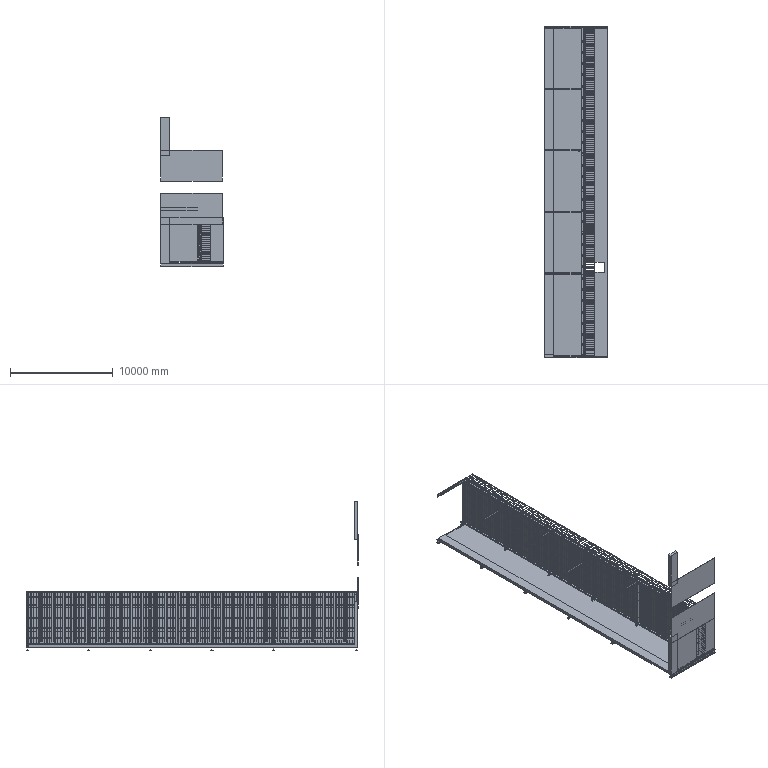Assembly | SolidWorks | mm | 472 component files | 530 solids | 11239 faces | box 6100 x 32341.42 x 14577.61 mm | volume 24746650782 mm3 | plane 7610 | cylinder 3629 | commonest cylinder face diameters 12 x1644 6 x1644 26 x76 2.667 x70 10 x58 20 x58 56 x44 14 x35
Bill of materials:
30X30X3-1100 | 16 |  | Long straight square hollow tube with rounded outer and inner corners and a uniform wall.
30X30X3-940 | 162 |  | Long straight square hollow tube with rounded corners and a uniform wall.
63#AngleIron | 20 |  | Long angle (L-section) profile with legs of roughly equal length, a root fillet and slightly rounded leg tips. A narrow gap splits the length into two collinear pieces.
8mTread | 4 |  | Thin flat rectangular plate or strip with no visible holes or edge features.
ChannelSteel | 29 |  | Long straight channel (C-section) with sloped inner flange faces, root fillets between web and flanges, and rounded flange tips.
ColorSteelTile | 1 |  | Thin sheet-metal-like strip with one end bent up 90 degrees into a flange, giving an L-shaped side profile. The flat part has one rectangular cutout and a row of small slots or holes along its length.
Corbel | 5 |  | Short piece of wide-flange H/I-section with parallel flanges, a central web and large root fillets.
H200X100-3600 | 6 |  | Long I-section beam that is deep relative to its flange width, with a thin web, thin parallel flanges and root fillets.
H250X125-3800 | 5 |  | Long, slender H-section member with wide parallel flanges, a thin web and root fillets.
H250X125-7375 | 8 |  | Long H-section profile with wide flanges, a thin web and root fillets. It is shown lying with the web horizontal, so it looks like a trough in the isometric view.
Mirror30X30X3-940 | 159 |  | Long straight square hollow tube with rounded corners and a uniform wall.
Mirror30X30X3-1100 | 14 |  | Long straight square hollow tube with rounded corners and a uniform wall.
Mirror30X30X3-7440 | 8 |  | Long, slender straight tube with a square hollow cross-section and rounded corners. The length shows small breaks or seams, so it looks like three collinear lengths.
Mirror30X30X3-3720-30 | 2 |  | Straight square hollow tube with rounded corners, shown as a long thin member with breaks or seams dividing it into three collinear segments.
OriginalColumn | 6 |  | Straight I-section beam (wide-flange-like profile) with a constant cross-section along its length.
30X30X3-3720-30 | 2 |  | Straight square hollow tube with rounded corners, shown as a long thin member with breaks or seams dividing it into three collinear segments.
30X30X3-7440 | 8 |  | Long, slender straight tube with a square hollow cross-section and rounded corners. The length shows small breaks or seams, so it looks like three collinear lengths.
Tread | 16 |  | Thin flat rectangular plate or sheet with no visible holes or cutouts.
Wall | 1 |  | L-shaped arrangement of thin flat bars: a long horizontal strip joined at one end to a short upright strip. Two rectangular plates, separated by a gap, project sideways from the upright.
Mates:
1. width | H250X125-3800-1 face at (2060.926, 805.154, 99) dir (0, -1, 0) | H250X125-3800-1 face at (2069.926, 930.154, 99) dir (0, 1, 0) | OriginalColumn-1 face at (4369.926, 977.654, -147.679) dir (0, 1, 0) | OriginalColumn-1 face at (4369.926, 757.654, -167.679) dir (0, -1, 0)
2. coincident | H200X100-3600-1 face at (1819.926, 851.904, 5050) dir (1, 0, 0) | H250X125-3800-1 face at (1819.926, 930.154, 99) dir (-1, 0, 0)
3. width | H200X100-3600-1 face at (1819.926, 805.154, 5029) dir (0, -1, 0) | H200X100-3600-1 face at (1819.926, 930.154, 5037) dir (0, 1, 0) | H250X125-3800-1 face at (1828.926, 930.154, 99) dir (0, 1, 0) | H250X125-3800-1 face at (1819.926, 805.154, 99) dir (0, -1, 0)
4. coincident | H200X100-3600-1 face at (1819.926, 805.154, 5279) dir (0, 0, 1) | H250X125-3800-1 face at (1841.926, 851.654, 5279) dir (0, 0, 1)
5. coincident | H250X125-3800-1 face at (2069.926, 805.154, 99) dir (1, 0, 0) | H250X125-7375-1 face at (2069.926, 805.154, 5154) dir (1, 0, 0)
6. coincident | H250X125-3800-1 face at (1819.926, 805.154, 99) dir (0, -1, 0) | H250X125-7375-1 face at (1841.926, 805.154, 5200.5) dir (0, 1, 0)
7. distance | ChannelSteel-1 face at (1912.304, -394.846, 164.5) dir (0, 1, 0) | H250X125-3800-1 face at (2060.926, 805.154, 99) dir (0, -1, 0)
8. coincident | H250X125-3800-1 face at (2069.926, 805.154, 99) dir (1, 0, 0) | 63#AngleIron-1 face at (2069.926, 805.154, 4696) dir (1, 0, 0)
9. coincident | H250X125-3800-1 face at (2060.926, 805.154, 99) dir (0, -1, 0) | 63#AngleIron-1 face at (2008.259, 805.154, 4756.333) dir (0, 1, 0)
10. coincident | H250X125-3800-1 face at (2069.926, 805.154, 99) dir (1, 0, 0) | assembly face at (2069.774, 874.154, 4042) dir (-1, 0, 0)
11. distance | assembly face at (3169.774, 880.154, 4042) dir (0, 1, 0) | H250X125-3800-1 face at (2069.926, 930.154, 99) dir (0, 1, 0)
12. distance | assembly face at (3169.774, 874.154, 4048) dir (0, 0, 1) | H250X125-3800-1 face at (1841.926, 851.654, 5279) dir (0, 0, 1)
13. coincident | ChannelSteel-1 face at (1912.304, -594.846, 164.5) dir (1, 0, 0) | Floor-1 face at (2069.774, 930.154, 2588) dir (-1, 0, 0)
14. coincident | H250X125-7375-1 face at (2069.926, 805.154, 5279) dir (0, 0, 1) | Floor-1 face at (2069.774, 930.154, 4098) dir (0, 0, 1)
15. coincident | H250X125-3800-1 face at (2069.926, 930.154, 99) dir (0, 1, 0) | Floor-1 face at (2069.774, 930.154, 2588) dir (0, 1, 0)
16. coincident | assembly face at (3169.774, 880.154, 4042) dir (0, 1, 0) | assembly face at (3169.774, 880.154, 322) dir (0, -1, 0)
17. coincident | assembly face at (3169.774, 874.154, 4048) dir (0, 0, 1) | assembly face at (3169.774, 886.154, 4048) dir (0, 0, 1)
18. coincident | OriginalColumn-1 face at (4369.926, 757.654, -167.679) dir (0, -1, 0) | assembly face at (3169.774, 717.654, -128) dir (0, 1, 0)
19. distance | OriginalColumn-2 face at (4369.926, -5098.346, -167.679) dir (0, 0, -1) | assembly face at (3169.774, -6458.346, -122) dir (0, 0, 1)
20. coincident | Tread-1 face at (2069.926, 8778.376, -4819.381) dir (-1, 0, 0) | H250X125-7375-15 face at (2019.774, 805.154, 99) dir (1, 0, 0)
21. coincident | OriginalColumn-1 face at (4369.926, 757.654, -147.679) dir (0, 0, 1) | Corbel-1 face at (1771.926, 833.654, -147.679) dir (0, 0, -1)
22. width | OriginalColumn-1 face at (4369.926, 977.654, -147.679) dir (0, 1, 0) | OriginalColumn-1 face at (4369.926, 757.654, -167.679) dir (0, -1, 0) | Corbel-1 face at (1819.926, 805.154, 352.321) dir (0, -1, 0) | Corbel-1 face at (1799.926, 930.154, 352.321) dir (0, 1, 0)
23. coincident | OriginalColumn-1 face at (-1730.074, 833.654, -449.679) dir (-1, 0, 0) | Wall-1 face at (-1730.074, 4663.226, -160.714) dir (-1, 0, 0)
24. coincident | OriginalColumn-1 face at (4369.926, 757.654, -147.679) dir (0, 0, 1) | Wall-1 face at (-830.074, 757.654, -147.679) dir (0, 0, -1)
25. distance | H250X125-7375-15 face at (2010.774, 805.154, 99) dir (0, 0, -1) | Tread-1 face at (2069.926, 890.154, 139) dir (0, 0, -1)
26. distance | H250X125-7375-16 face at (1841.926, 805.154, 158.5) dir (0, 0, -1) | OriginalColumn-1 face at (4369.926, 757.654, -147.679) dir (0, 0, 1)
27. distance | H250X125-3800-1 face at (1841.926, 851.654, 99) dir (0, 0, -1) | Tread-1 face at (2069.926, 890.154, 139) dir (0, 0, -1)
28. coincident | Railing-2-2/30X30X3-1100-3 face at (3169.926, -31194.846, 3843) dir (0, -1, 0) | 30X30X3-1100-3 face at (3169.926, -31194.846, 5273) dir (0, -1, 0)
29. coincident | Railing-2-2/30X30X3-3720-30-1 face at (3163.926, -31170.846, 5249) dir (0, 0, 1) | 30X30X3-1100-3 face at (3169.926, -31170.846, 5249) dir (0, 0, -1)
30. coincident | Railing-2-2/30X30X3-3720-30-1 face at (3169.926, -31170.846, 5249) dir (1, 0, 0) | 30X30X3-1100-3 face at (3169.926, -31170.846, 5255) dir (1, 0, 0)
31. coincident | Railing-2-2/30X30X3-940-16 face at (3139.926, -31194.846, 3648) dir (0, -1, 0) | 30X30X3-940-1 face at (3139.926, -31194.846, 3908) dir (0, -1, 0)
32. coincident | Railing-2-2/30X30X3-3720-30-2 face at (2199.926, -31170.846, 5249) dir (1, 0, 0) | 30X30X3-940-1 face at (2199.926, -31170.846, 3890) dir (-1, 0, 0)
33. coincident | H200X100-3600-6 face at (-1730.074, -29148.096, 5050) dir (-1, 0, 0) | Wall-1 face at (-1730.074, 4663.226, -160.714) dir (-1, 0, 0)
34. coincident | Tread-1 face at (2069.926, 8778.376, -4819.381) dir (-1, 0, 0) | H250X125-7375-16 face at (2069.926, 805.154, 99) dir (1, 0, 0)
35. lock | H250X125-3800-6 reference at (0, 0, 0) dir (1, 0, 0) | 30X30X3-1100-3 reference at (0, 0, 0) dir (1, 0, 0)
36. coincident | H250X125-3800-1 face at (2069.926, 805.154, 99) dir (1, 0, 0) | Railing-6/30X30X3-1100-1 face at (2069.926, 922.294, 5273) dir (-1, 0, 0)
37. coincident | H250X125-7375-4 face at (2069.926, -23194.846, 5154) dir (1, 0, 0) | 30X30X3-1100-3 face at (2069.926, -31170.846, 5255) dir (-1, 0, 0)
38. coincident | H250X125-7375-4 face at (2069.926, -23194.846, 5279) dir (0, 0, 1) | 30X30X3-1100-3 face at (3169.926, -31188.846, 5279) dir (0, 0, 1)
39. coincident | H250X125-7375-4 face at (1841.926, -31194.846, 5200.5) dir (0, -1, 0) | 30X30X3-1100-3 face at (3169.926, -31194.846, 5273) dir (0, -1, 0)
40. coincident | Railing-6/30X30X3-1100-3 face at (3169.926, -6547.706, 5279) dir (0, 0, 1) | 30X30X3-940-6 face at (3139.926, -6811.197, 5279) dir (0, 0, 1)
41. lock | H250X125-7375-4 reference at (0, 0, 0) dir (1, 0, 0) | 30X30X3-1100-3 reference at (0, 0, 0) dir (1, 0, 0)
42. coincident | H250X125-7375-19 face at (2069.926, -23194.846, 99) dir (1, 0, 0) | 8mTread-1 face at (2069.926, -13426.79, -4794.447) dir (-1, 0, 0)
43. coincident | Tread-76 edge at (2077.926, -17139.846, 139) dir (0, -1, 0) | 8mTread-1 edge at (2077.926, -23149.846, 139) dir (0, -1, 0)
44. distance | Tread-76 face at (2069.926, -23139.846, 139) dir (0, -1, 0) | 8mTread-1 face at (2069.926, -23149.846, 139) dir (0, 1, 0)
45. distance | H250X125-3800-1 face at (1841.926, 851.654, 99) dir (0, 0, -1) | ChannelSteel-1 vertex at (1894.378, -405.685, 164.5) dir (1, 0, 0)
46. lock | H250X125-3800-1 reference at (0, 0, 0) dir (1, 0, 0) | Railing-6/30X30X3-1100-1 reference at (0, 0, 0) dir (1, 0, 0)
47. lock | Railing-6/30X30X3-7440-1 reference at (0, 0, 0) dir (1, 0, 0) | 30X30X3-940-6 reference at (0, 0, 0) dir (1, 0, 0)
48. coincident | Mirror30X30X3-1100-1 face at (-381.487, 603.212, -30) dir (0, 0, -1) | Mirror30X30X3-7440-1 face at (7642.513, 597.212, -30) dir (0, 0, -1)
49. coincident | Mirror30X30X3-1100-1 face at (-357.487, 603.212, -6) dir (1, 0, 0) | Mirror30X30X3-7440-1 face at (-357.487, 597.212, -24) dir (-1, 0, 0)
50. coincident | Mirror30X30X3-1100-1 face at (-381.487, 603.212, -24) dir (0, 1, 0) | Mirror30X30X3-7440-1 face at (7642.513, 603.212, -24) dir (0, 1, 0)
51. coincident | Mirror30X30X3-1100-1 face at (-381.487, 603.212, -30) dir (0, 0, -1) | Mirror30X30X3-940-1 face at (-171.487, 573.212, -30) dir (0, 0, -1)
52. coincident | Mirror30X30X3-7440-1 face at (7642.513, 573.212, -6) dir (0, -1, 0) | Mirror30X30X3-940-1 face at (-171.487, 573.212, -24) dir (0, 1, 0)
53. coincident | Mirror30X30X3-1100-1 face at (-381.487, 603.212, -30) dir (0, 0, -1) | Mirror30X30X3-7440-2 face at (7642.513, -372.788, -30) dir (0, 0, -1)
54. coincident | Mirror30X30X3-1100-1 face at (-357.487, 603.212, -6) dir (1, 0, 0) | Mirror30X30X3-7440-2 face at (-357.487, -372.788, -24) dir (-1, 0, 0)
55. coincident | Mirror30X30X3-940-1 face at (-171.487, -366.788, -24) dir (0, -1, 0) | Mirror30X30X3-7440-2 face at (7642.513, -366.788, -24) dir (0, 1, 0)
56. distance | Mirror30X30X3-940-1 face at (-177.487, 573.212, -24) dir (-1, 0, 0) | Mirror30X30X3-1100-1 face at (-357.487, 603.212, -6) dir (1, 0, 0)
57. coincident | Mirror30X30X3-1100-1 face at (-381.487, 603.212, -30) dir (0, 0, -1) | Mirror30X30X3-7440-1 face at (7642.513, 597.212, -30) dir (0, 0, -1)
58. coincident | Mirror30X30X3-1100-1 face at (-357.487, 603.212, -6) dir (1, 0, 0) | Mirror30X30X3-7440-1 face at (-357.487, 597.212, -24) dir (-1, 0, 0)
59. coincident | Mirror30X30X3-1100-1 face at (-381.487, 603.212, -24) dir (0, 1, 0) | Mirror30X30X3-7440-1 face at (7642.513, 603.212, -24) dir (0, 1, 0)
60. coincident | Mirror30X30X3-1100-1 face at (-381.487, 603.212, -30) dir (0, 0, -1) | Mirror30X30X3-940-1 face at (-171.487, 573.212, -30) dir (0, 0, -1)
61. coincident | Mirror30X30X3-7440-1 face at (7642.513, 573.212, -6) dir (0, -1, 0) | Mirror30X30X3-940-1 face at (-171.487, 573.212, -24) dir (0, 1, 0)
62. coincident | Mirror30X30X3-1100-1 face at (-381.487, 603.212, -30) dir (0, 0, -1) | Mirror30X30X3-7440-2 face at (7642.513, -372.788, -30) dir (0, 0, -1)
63. coincident | Mirror30X30X3-1100-1 face at (-357.487, 603.212, -6) dir (1, 0, 0) | Mirror30X30X3-7440-2 face at (-357.487, -372.788, -24) dir (-1, 0, 0)
64. coincident | Mirror30X30X3-940-1 face at (-171.487, -366.788, -24) dir (0, -1, 0) | Mirror30X30X3-7440-2 face at (7642.513, -366.788, -24) dir (0, 1, 0)
65. distance | Mirror30X30X3-940-1 face at (-177.487, 573.212, -24) dir (-1, 0, 0) | Mirror30X30X3-1100-1 face at (-357.487, 603.212, -6) dir (1, 0, 0)
66. coincident | Mirror30X30X3-1100-1 face at (-381.487, 603.212, -30) dir (0, 0, -1) | Mirror30X30X3-7440-1 face at (7642.513, 597.212, -30) dir (0, 0, -1)
67. coincident | Mirror30X30X3-1100-1 face at (-357.487, 603.212, -6) dir (1, 0, 0) | Mirror30X30X3-7440-1 face at (-357.487, 597.212, -24) dir (-1, 0, 0)
68. coincident | Mirror30X30X3-1100-1 face at (-381.487, 603.212, -24) dir (0, 1, 0) | Mirror30X30X3-7440-1 face at (7642.513, 603.212, -24) dir (0, 1, 0)
69. coincident | Mirror30X30X3-1100-1 face at (-381.487, 603.212, -30) dir (0, 0, -1) | Mirror30X30X3-940-1 face at (-171.487, 573.212, -30) dir (0, 0, -1)
70. coincident | Mirror30X30X3-7440-1 face at (7642.513, 573.212, -6) dir (0, -1, 0) | Mirror30X30X3-940-1 face at (-171.487, 573.212, -24) dir (0, 1, 0)
71. coincident | Mirror30X30X3-1100-1 face at (-381.487, 603.212, -30) dir (0, 0, -1) | Mirror30X30X3-7440-2 face at (7642.513, -372.788, -30) dir (0, 0, -1)
72. coincident | Mirror30X30X3-1100-1 face at (-357.487, 603.212, -6) dir (1, 0, 0) | Mirror30X30X3-7440-2 face at (-357.487, -372.788, -24) dir (-1, 0, 0)
73. coincident | Mirror30X30X3-940-1 face at (-171.487, -366.788, -24) dir (0, -1, 0) | Mirror30X30X3-7440-2 face at (7642.513, -366.788, -24) dir (0, 1, 0)
74. distance | Mirror30X30X3-940-1 face at (-177.487, 573.212, -24) dir (-1, 0, 0) | Mirror30X30X3-1100-1 face at (-357.487, 603.212, -6) dir (1, 0, 0)
75. coincident | Mirror30X30X3-1100-1 face at (-381.487, 603.212, -30) dir (0, 0, -1) | Mirror30X30X3-7440-1 face at (7642.513, 597.212, -30) dir (0, 0, -1)
76. coincident | Mirror30X30X3-1100-1 face at (-357.487, 603.212, -6) dir (1, 0, 0) | Mirror30X30X3-7440-1 face at (-357.487, 597.212, -24) dir (-1, 0, 0)
77. coincident | Mirror30X30X3-1100-1 face at (-381.487, 603.212, -24) dir (0, 1, 0) | Mirror30X30X3-7440-1 face at (7642.513, 603.212, -24) dir (0, 1, 0)
78. coincident | Mirror30X30X3-1100-1 face at (-381.487, 603.212, -30) dir (0, 0, -1) | Mirror30X30X3-940-1 face at (-171.487, 573.212, -30) dir (0, 0, -1)
79. coincident | Mirror30X30X3-7440-1 face at (7642.513, 573.212, -6) dir (0, -1, 0) | Mirror30X30X3-940-1 face at (-171.487, 573.212, -24) dir (0, 1, 0)
80. coincident | Mirror30X30X3-1100-1 face at (-381.487, 603.212, -30) dir (0, 0, -1) | Mirror30X30X3-7440-2 face at (7642.513, -372.788, -30) dir (0, 0, -1)
81. coincident | Mirror30X30X3-1100-1 face at (-357.487, 603.212, -6) dir (1, 0, 0) | Mirror30X30X3-7440-2 face at (-357.487, -372.788, -24) dir (-1, 0, 0)
82. coincident | Mirror30X30X3-940-1 face at (-171.487, -366.788, -24) dir (0, -1, 0) | Mirror30X30X3-7440-2 face at (7642.513, -366.788, -24) dir (0, 1, 0)
83. distance | Mirror30X30X3-940-1 face at (-177.487, 573.212, -24) dir (-1, 0, 0) | Mirror30X30X3-1100-1 face at (-357.487, 603.212, -6) dir (1, 0, 0)
84. coincident | Mirror30X30X3-3720-30-1 face at (-348.618, 682.943, -24) dir (-1, 0, 0) | Mirror30X30X3-3720-30-2 face at (-348.618, -287.057, -24) dir (-1, 0, 0)
85. coincident | Mirror30X30X3-3720-30-1 face at (4771.382, 688.943, -24) dir (0, 1, 0) | Mirror30X30X3-1100-2 face at (1487.382, 688.943, -24) dir (0, 1, 0)
86. coincident | Mirror30X30X3-940-1 face at (-162.618, 658.943, -30) dir (0, 0, -1) | Mirror30X30X3-1100-2 face at (1487.382, 688.943, -30) dir (0, 0, -1)
87. coincident | Mirror30X30X3-1100-2 face at (1487.382, 688.943, -30) dir (0, 0, -1) | Mirror30X30X3-3720-30-2 face at (4771.382, -287.057, -30) dir (0, 0, -1)
88. distance | Mirror30X30X3-1100-2 face at (1481.382, 688.943, -24) dir (-1, 0, 0) | Mirror30X30X3-3720-30-2 face at (-348.618, -287.057, -24) dir (-1, 0, 0)
89. distance | Mirror30X30X3-3720-30-2 face at (-348.618, -287.057, -24) dir (-1, 0, 0) | Mirror30X30X3-940-1 face at (-168.618, 658.943, -24) dir (-1, 0, 0)
90. coincident | 30X30X3-1100-1 face at (-348.618, 688.943, 6) dir (1, 0, 0) | 30X30X3-3720-30-1 face at (-348.618, 682.943, 24) dir (-1, 0, 0)
91. coincident | 30X30X3-1100-1 face at (-372.618, 688.943, 24) dir (0, 1, 0) | 30X30X3-3720-30-1 face at (4771.382, 688.943, 24) dir (0, 1, 0)
92. coincident | 30X30X3-1100-1 face at (-372.618, 688.943, 30) dir (0, 0, 1) | 30X30X3-940-1 face at (-162.618, 658.943, 30) dir (0, 0, 1)
93. coincident | 30X30X3-3720-30-1 face at (4771.382, 658.943, 6) dir (0, -1, 0) | 30X30X3-940-1 face at (-162.618, 658.943, 24) dir (0, 1, 0)
94. coincident | 30X30X3-1100-1 face at (-372.618, 688.943, 30) dir (0, 0, 1) | 30X30X3-3720-30-2 face at (4771.382, -287.057, 30) dir (0, 0, 1)
95. coincident | 30X30X3-940-1 face at (-162.618, -281.057, 24) dir (0, -1, 0) | 30X30X3-3720-30-2 face at (4771.382, -281.057, 24) dir (0, 1, 0)
96. coincident | 30X30X3-1100-1 face at (-348.618, 688.943, 6) dir (1, 0, 0) | 30X30X3-3720-30-2 face at (-348.618, -287.057, 24) dir (-1, 0, 0)
97. distance | 30X30X3-1100-1 face at (-348.618, 688.943, 6) dir (1, 0, 0) | 30X30X3-940-1 face at (-168.618, 658.943, 24) dir (-1, 0, 0)
98. coincident | 30X30X3-1100-1 face at (-381.487, 603.212, 30) dir (0, 0, 1) | 30X30X3-7440-1 face at (7642.513, 597.212, 30) dir (0, 0, 1)
99. coincident | 30X30X3-1100-1 face at (-357.487, 603.212, 6) dir (1, 0, 0) | 30X30X3-7440-1 face at (-357.487, 597.212, 24) dir (-1, 0, 0)
100. coincident | 30X30X3-1100-1 face at (-381.487, 603.212, 24) dir (0, 1, 0) | 30X30X3-7440-1 face at (7642.513, 603.212, 24) dir (0, 1, 0)
101. coincident | 30X30X3-1100-1 face at (-381.487, 603.212, 30) dir (0, 0, 1) | 30X30X3-940-1 face at (-171.487, 573.212, 30) dir (0, 0, 1)
102. coincident | 30X30X3-7440-1 face at (7642.513, 573.212, 6) dir (0, -1, 0) | 30X30X3-940-1 face at (-171.487, 573.212, 24) dir (0, 1, 0)
103. coincident | 30X30X3-1100-1 face at (-381.487, 603.212, 30) dir (0, 0, 1) | 30X30X3-7440-2 face at (7642.513, -372.788, 30) dir (0, 0, 1)
104. coincident | 30X30X3-1100-1 face at (-357.487, 603.212, 6) dir (1, 0, 0) | 30X30X3-7440-2 face at (-357.487, -372.788, 24) dir (-1, 0, 0)
105. coincident | 30X30X3-940-1 face at (-171.487, -366.788, 24) dir (0, -1, 0) | 30X30X3-7440-2 face at (7642.513, -366.788, 24) dir (0, 1, 0)
106. distance | 30X30X3-940-1 face at (-177.487, 573.212, 24) dir (-1, 0, 0) | 30X30X3-1100-1 face at (-357.487, 603.212, 6) dir (1, 0, 0)